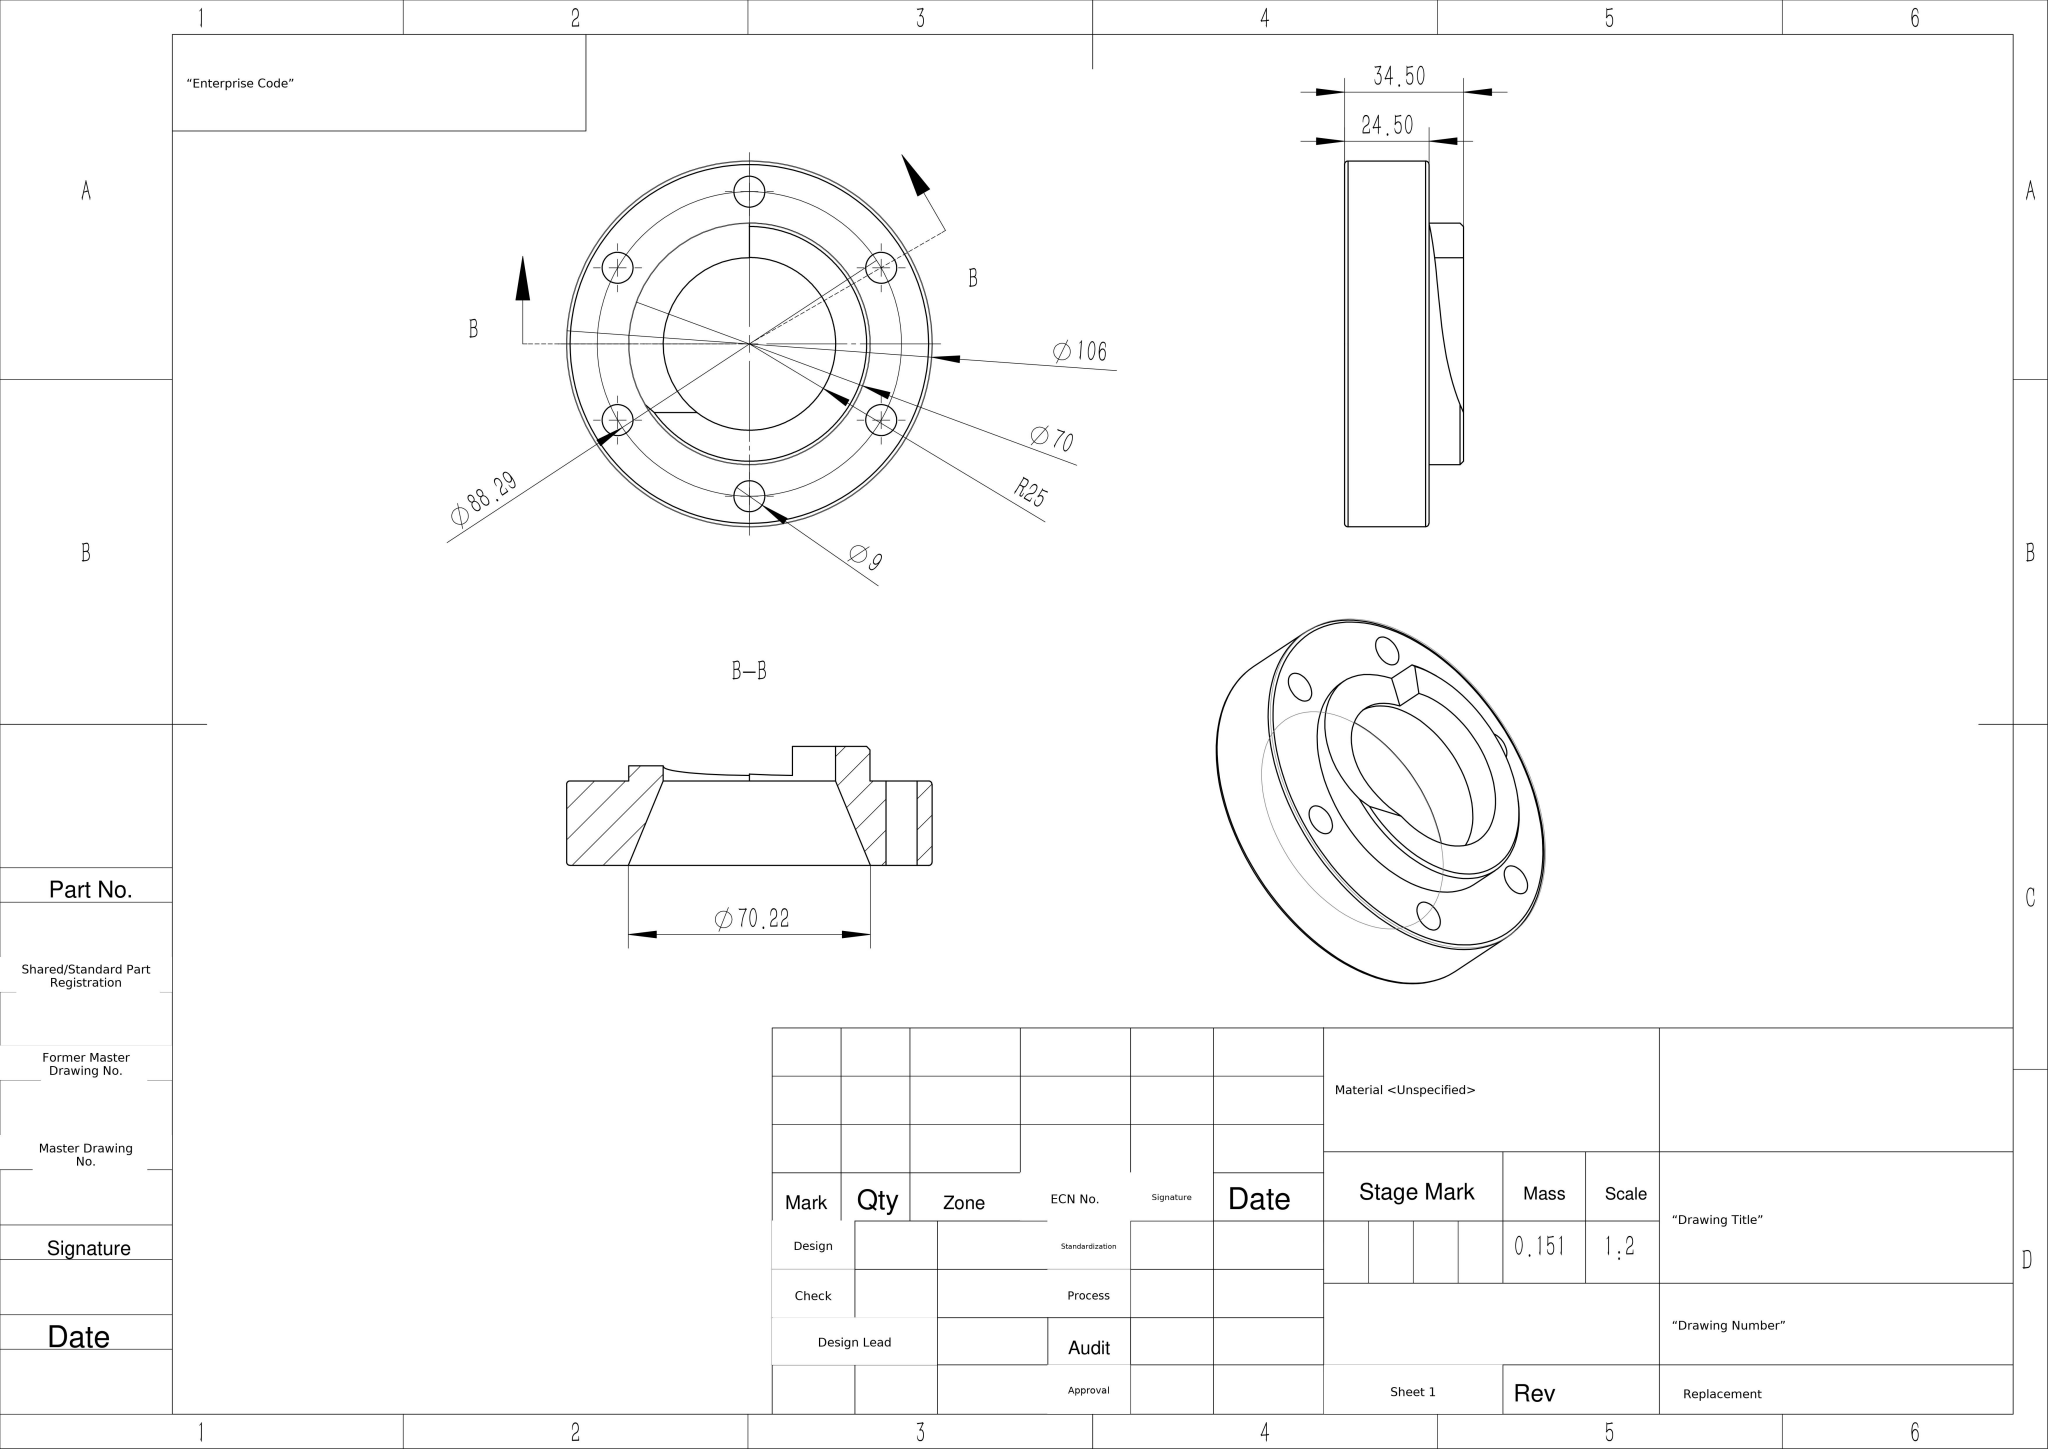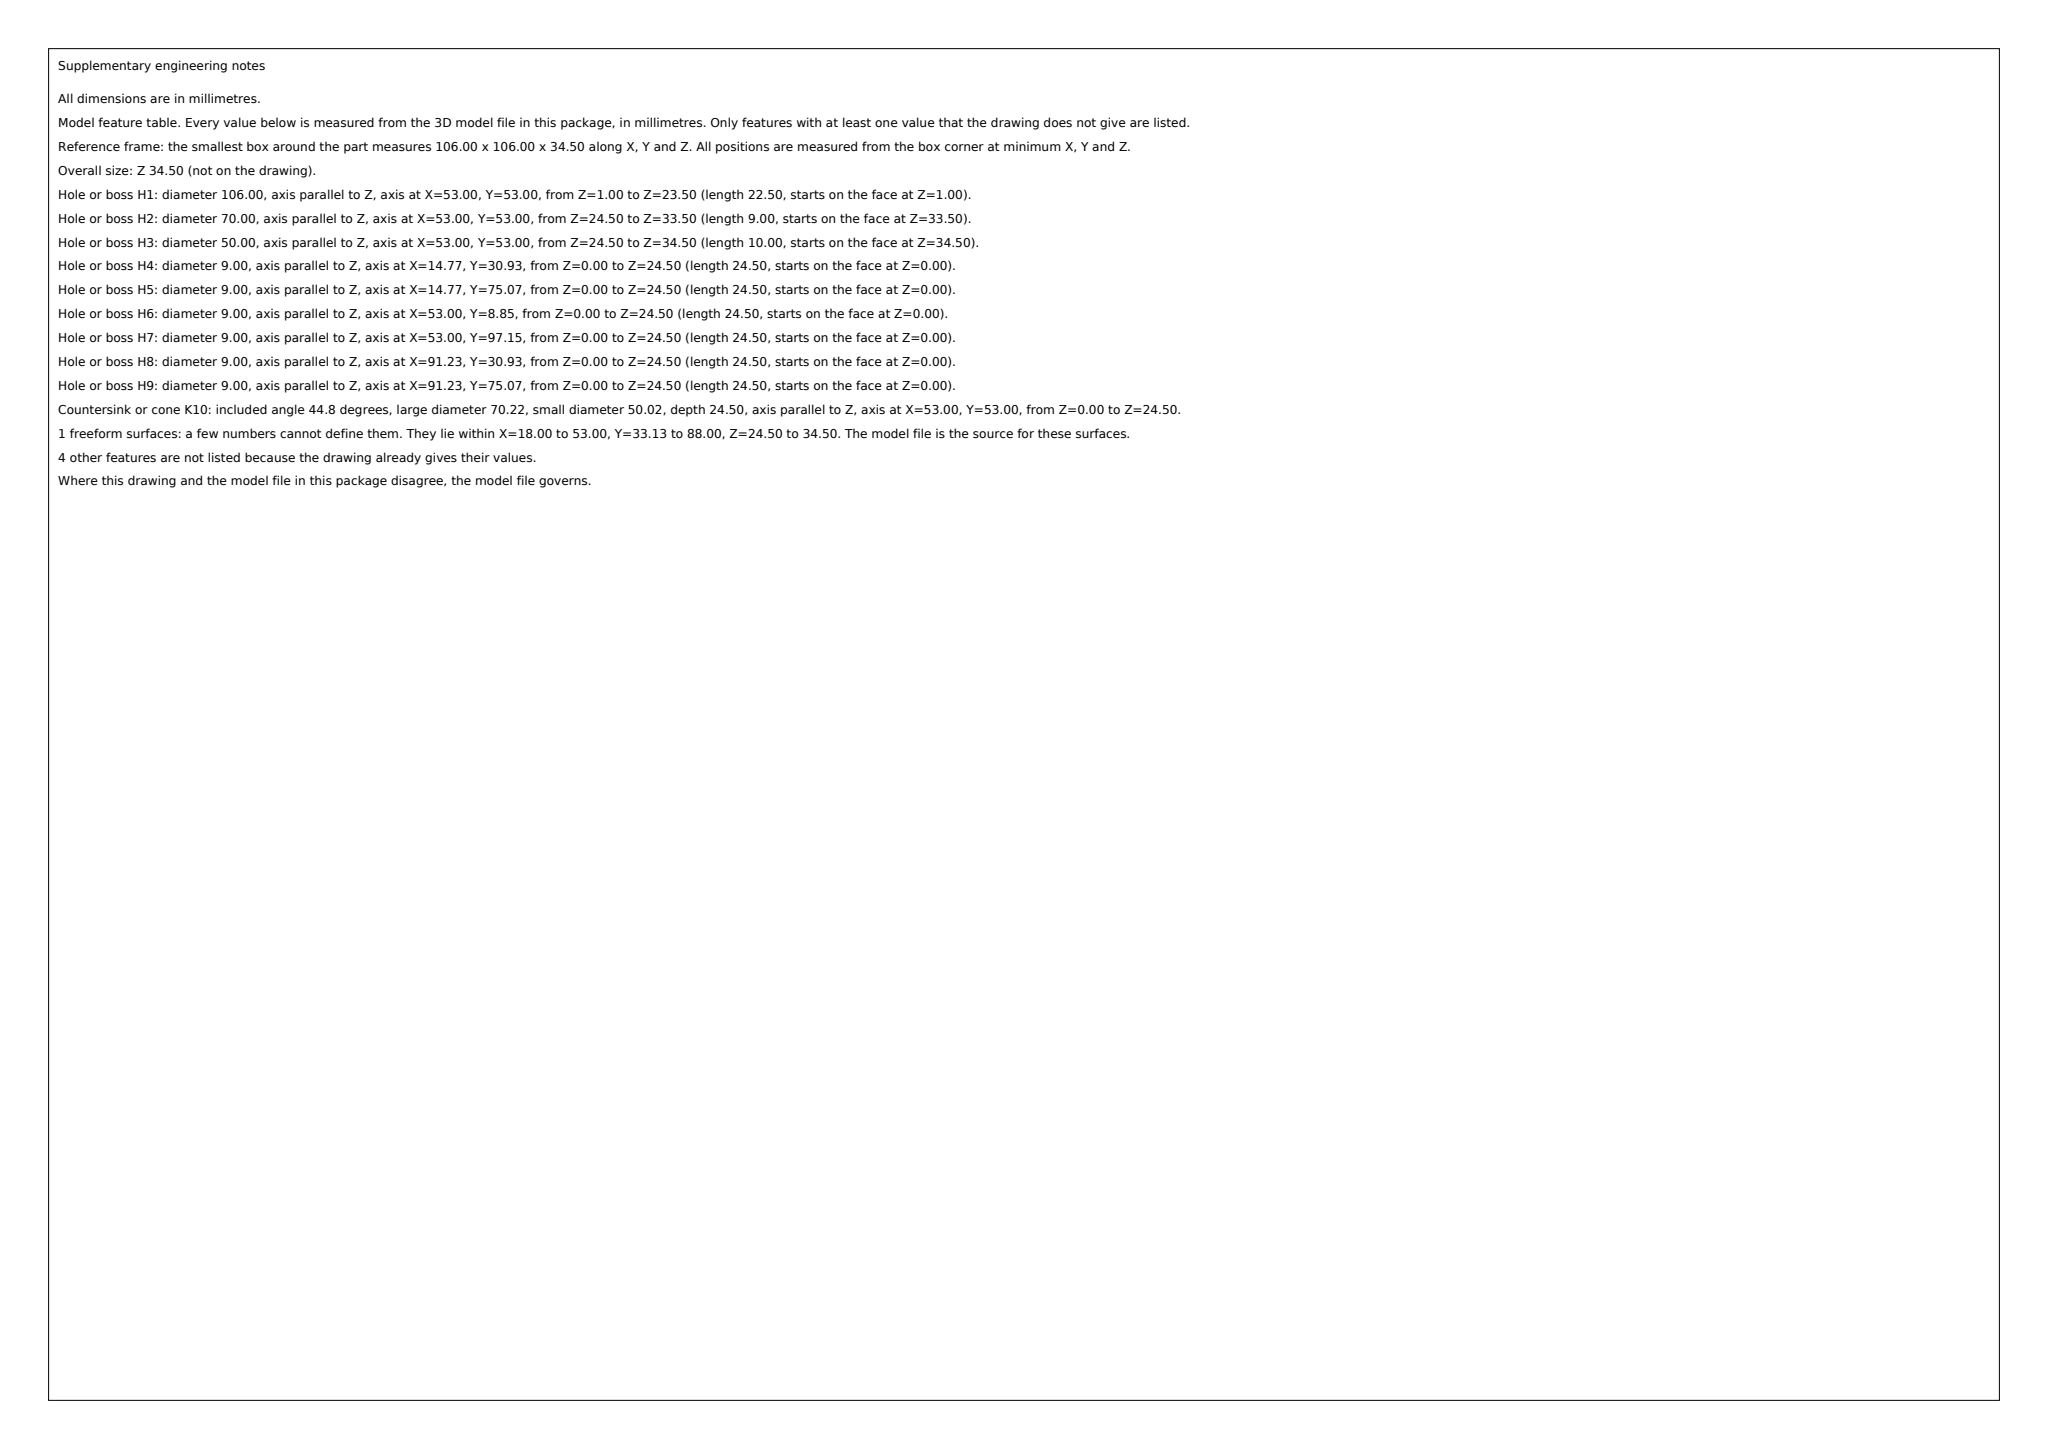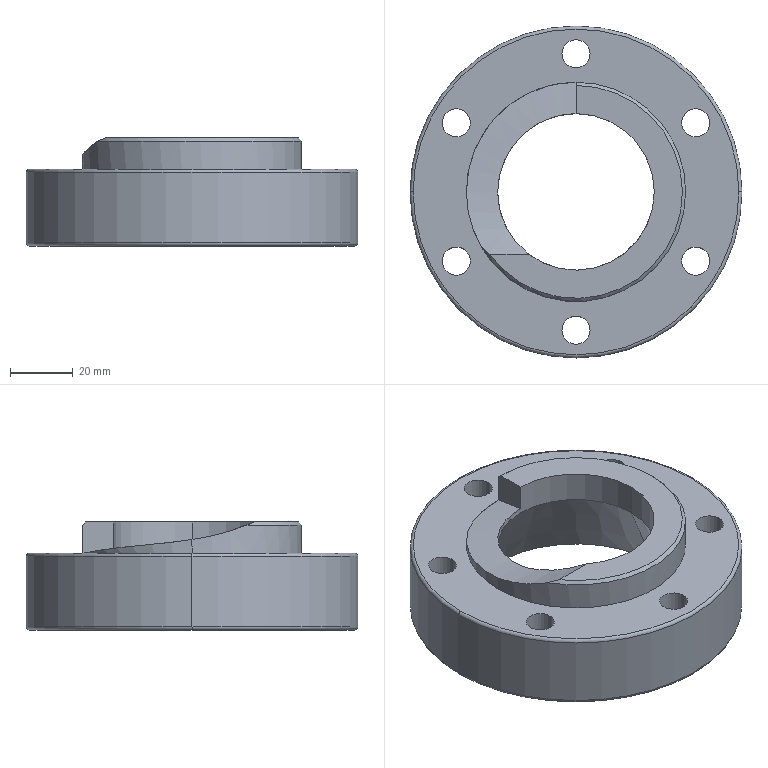Part | SolidWorks | mm | material <Unspecified> | 1 solid | 31 faces | box 106 x 106 x 34.5 mm | volume 150926 mm3 | cylinder 19 | torus 4 | plane 4 | cone 3 | spline 1 | commonest cylinder face diameters 9 x12 70 x3 106 x2 50 x2
build123d program:
from build123d import *
from build123d.topology import SkipClean

# Parameters (mm, degrees)
SKETCH1_R           = 35
SKETCH1_R_2         = 25
BOSS_EXTRUDE1_DEPTH = 10
SKETCH5_R           = 4.5
CUT_EXTRUDE1_DEPTH  = 64
CUT_EXTRUDE2_DEPTH  = 64
CHAMFER1_SIZE       = 1
FILLET3_R           = 1


with BuildPart() as part:
    # Sketch1 → Boss-Extrude1 (new body)
    with BuildSketch(Plane.XY):
        Circle(SKETCH1_R)
        Circle(SKETCH1_R_2, mode=Mode.SUBTRACT)
    extrude(amount=BOSS_EXTRUDE1_DEPTH)

    # Sketch4 → Revolve1 (revolve)
    with BuildSketch(Plane(origin=(0, 0, 0), x_dir=(1, 0, 0), z_dir=(0, 1, 0))):
        Polygon((53, 0), (53, 24.5), (35.109, 24.5), (25, 0), align=None)
    revolve(axis=Axis((0, 0, 0), (0, 0, -1)))

    # Sketch5 → Cut-Extrude1 (cut)
    with BuildSketch(Plane.XY):
        with Locations((0, 44.146)):
            Circle(SKETCH5_R)
        with Locations((38.231, 22.073)):
            Circle(SKETCH5_R)
        with Locations((38.231, -22.073)):
            Circle(SKETCH5_R)
        with Locations((0, -44.146)):
            Circle(SKETCH5_R)
        with Locations((-38.231, -22.073)):
            Circle(SKETCH5_R)
        with Locations((-38.231, 22.073)):
            Circle(SKETCH5_R)
    extrude(amount=-CUT_EXTRUDE1_DEPTH, mode=Mode.SUBTRACT)

    # Sketch7 → Cut-Extrude2 (cut)
    with SkipClean():  # the faces are left unmerged after this step: merging them gives an invalid solid
        with BuildSketch(Plane(origin=(0, 0, 0), x_dir=(0, 0, -1), z_dir=(1, 0, 0))):
            with BuildLine():
                Line((-14.52, 44.927), (0, 44.927))
                Line((0, 44.927), (0, 35))
                add(Edge.make_bspline(
                    [(0, 35), (-3.785, 16.786), (-2.073, -2.626), (-10, -19.869)],
                    knots=[0, 0, 0, 0, 1, 1, 1, 1], degree=3))
                Line((-10, -19.869), (-21.121, -19.869))
                Line((-21.121, -19.869), (-21.121, 44.927))
                Line((-21.121, 44.927), (-14.52, 44.927))
            make_face()
        extrude(amount=-CUT_EXTRUDE2_DEPTH, mode=Mode.SUBTRACT)

    # Chamfer1
    chamfer1_edges = [part.edges().sort_by_distance(p)[0] for p in [
        (10.405, -33.418, 10),
    ]]
    chamfer(chamfer1_edges, length=CHAMFER1_SIZE)

    # Fillet3
    fillet3_edges = [part.edges().sort_by_distance(p)[0] for p in [
        (-53, 0, -24.5),
        (-53, 0, 0),
    ]]
    fillet(fillet3_edges, radius=FILLET3_R)


solid = part.part